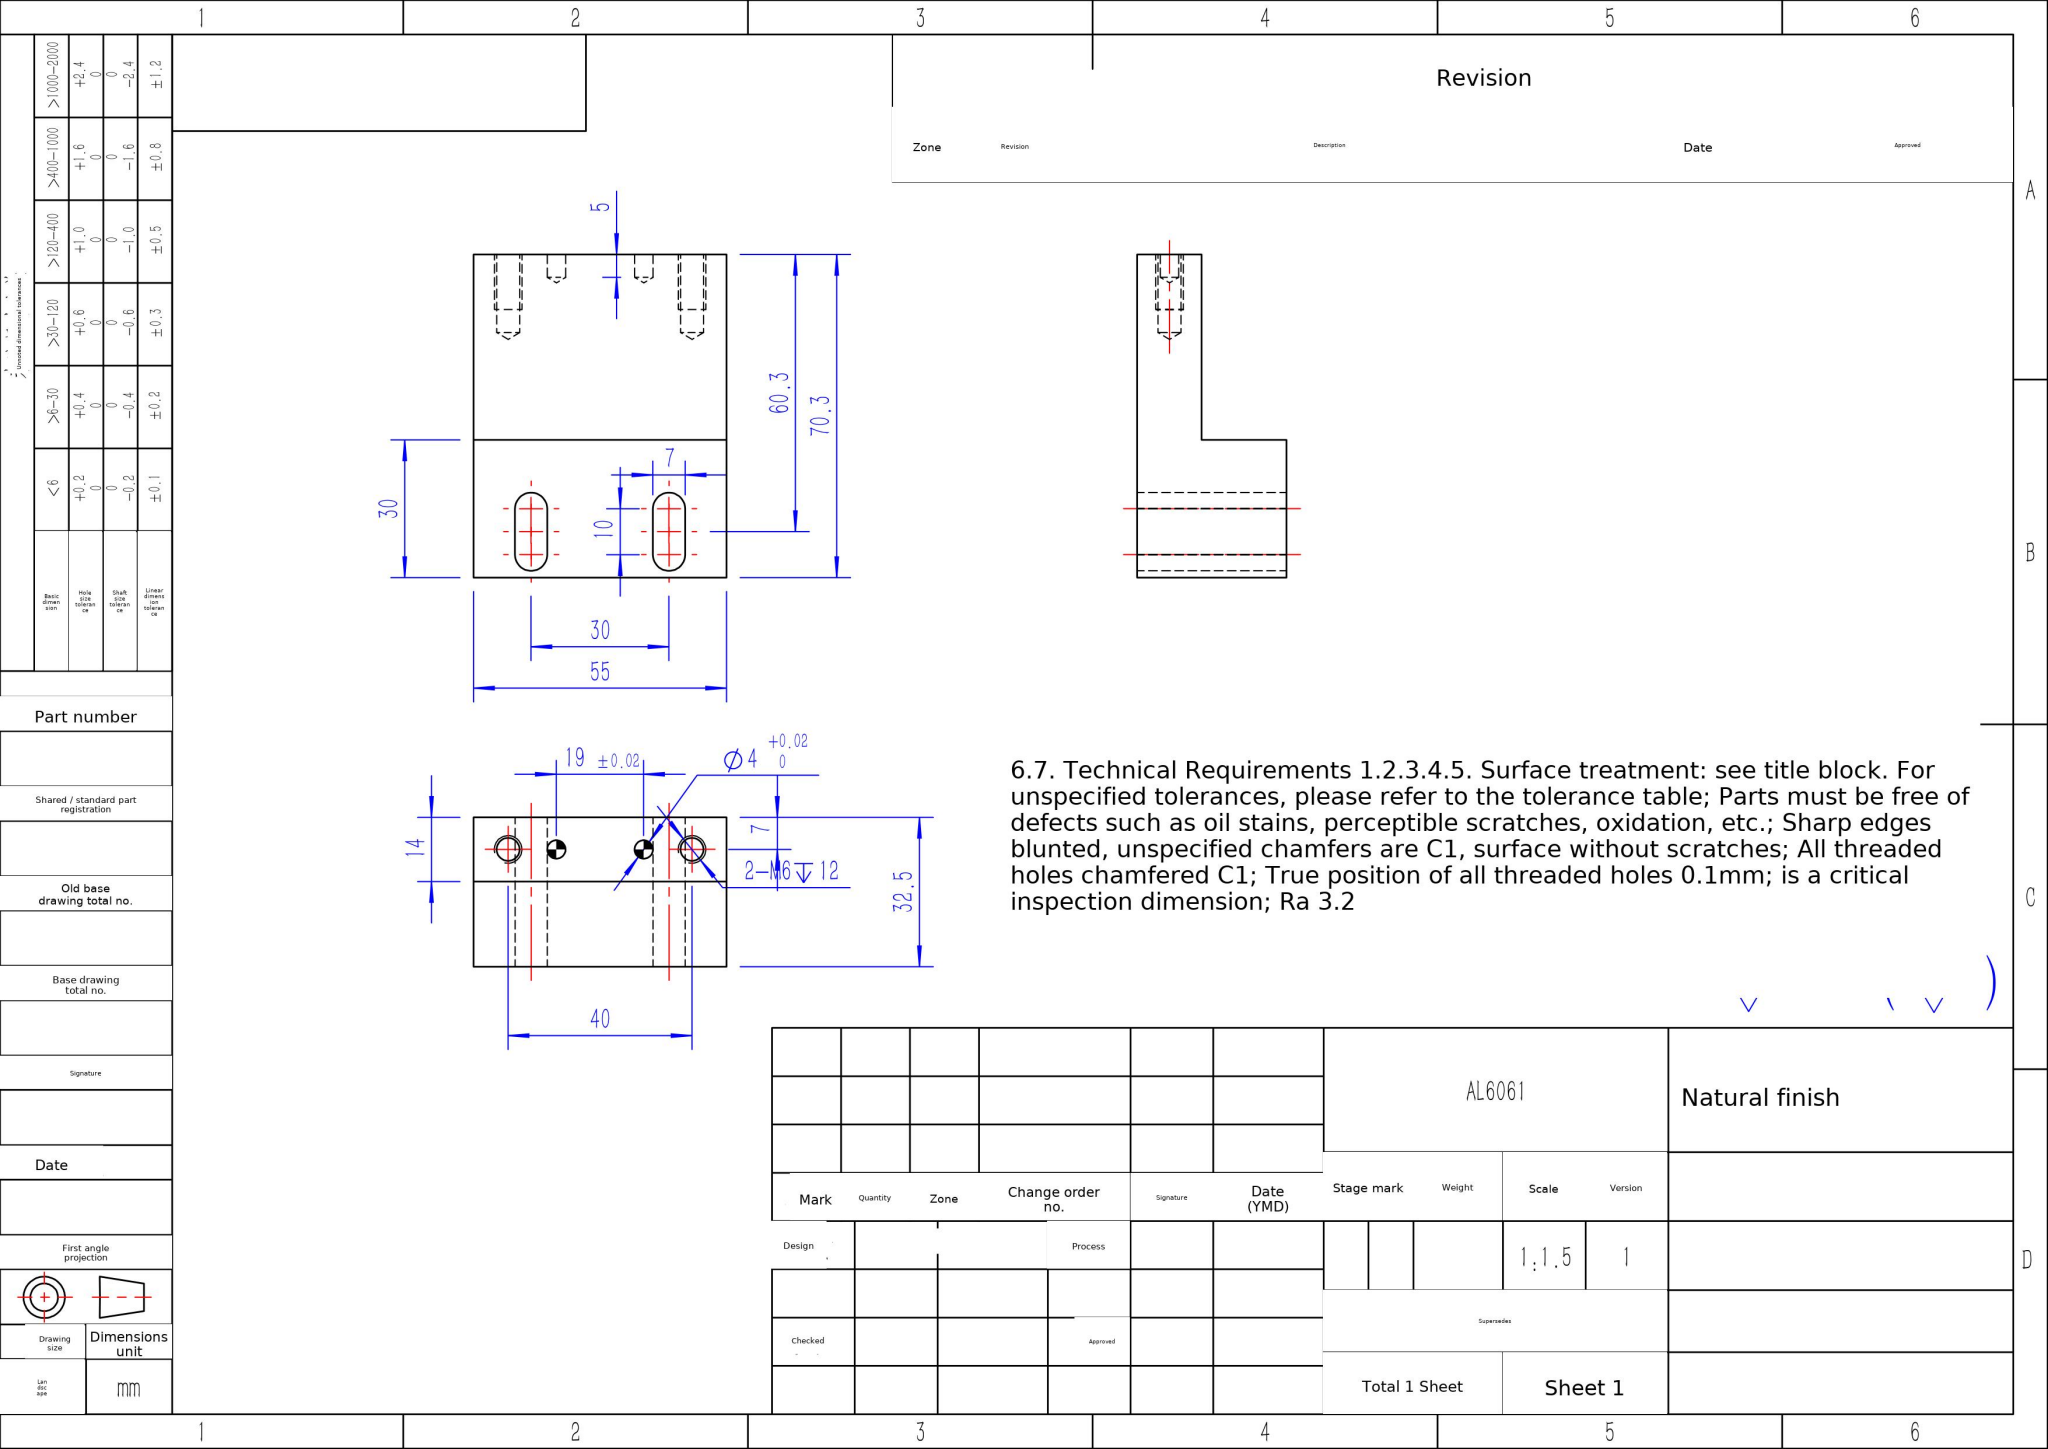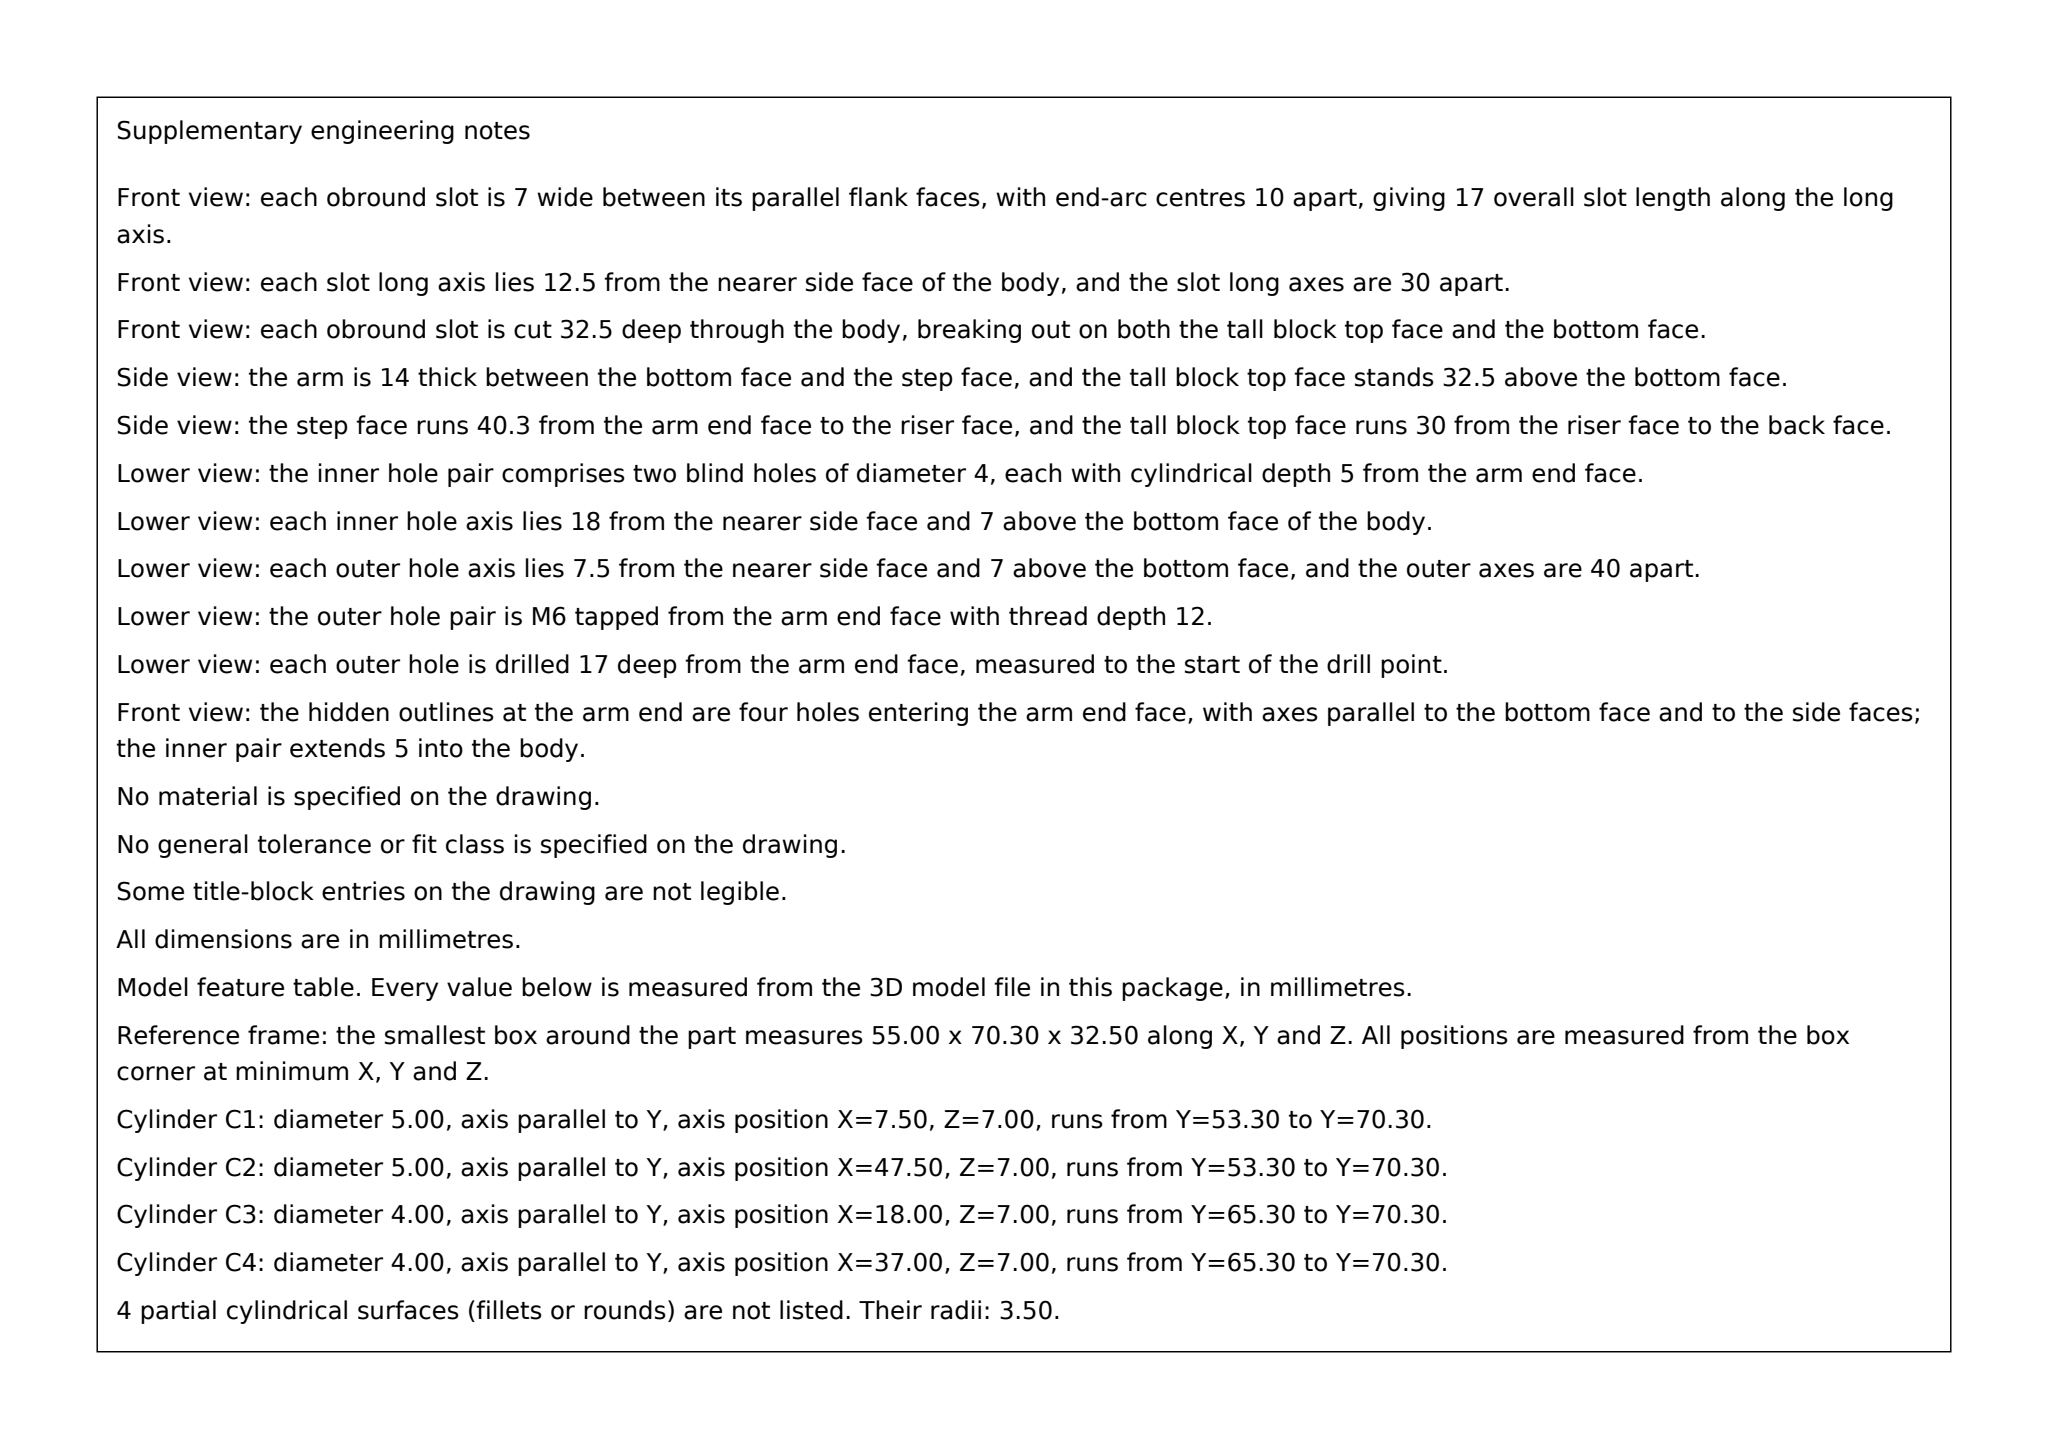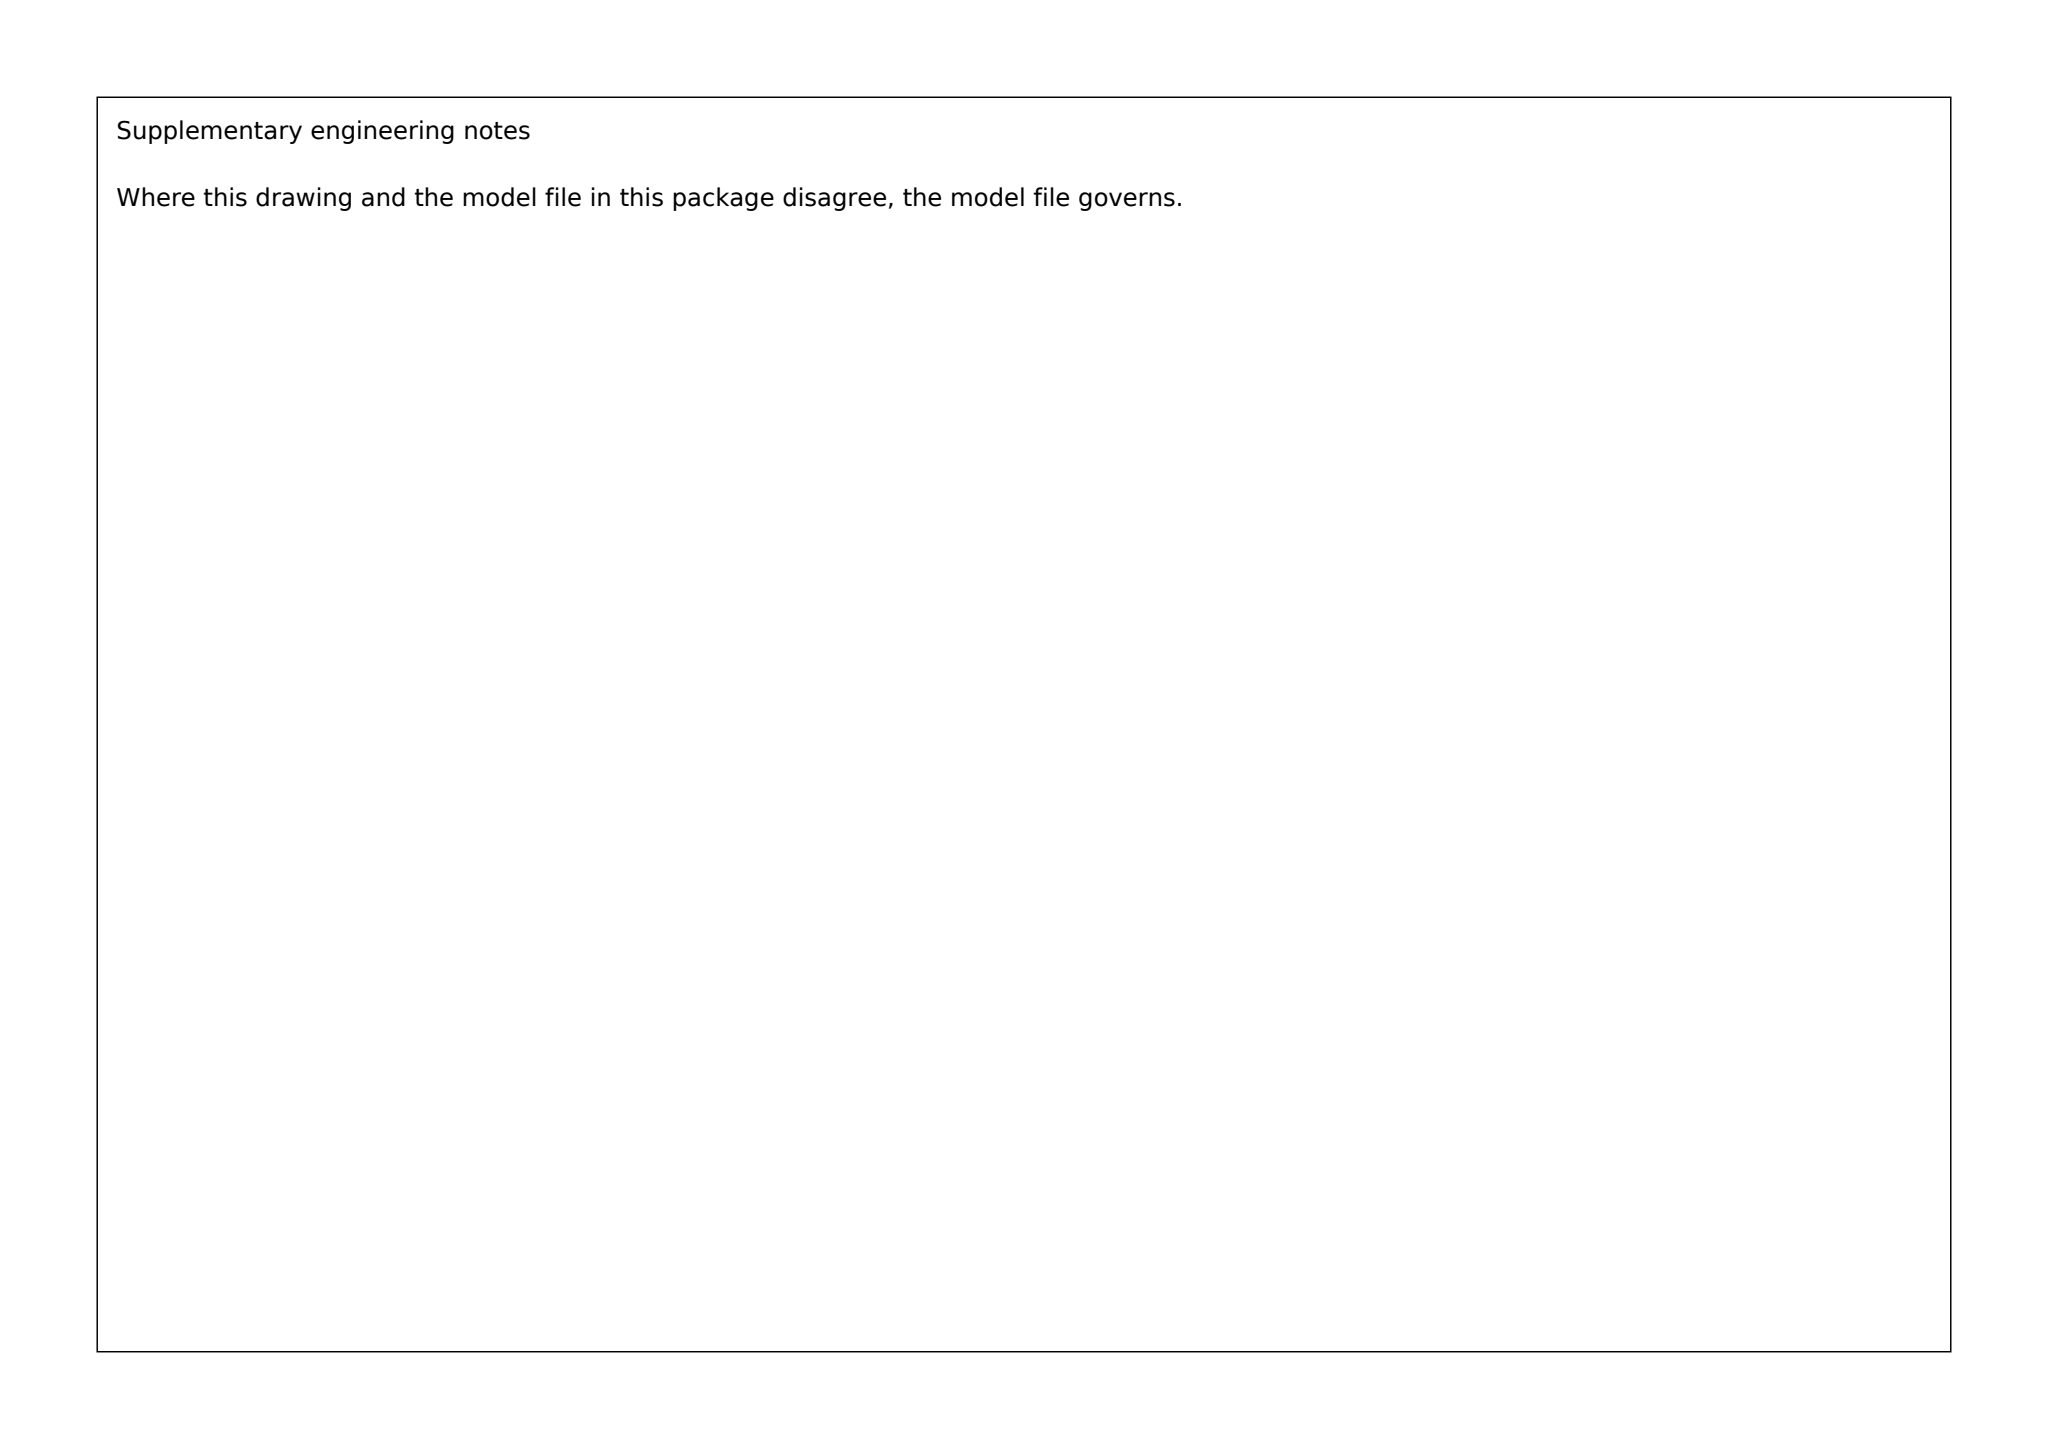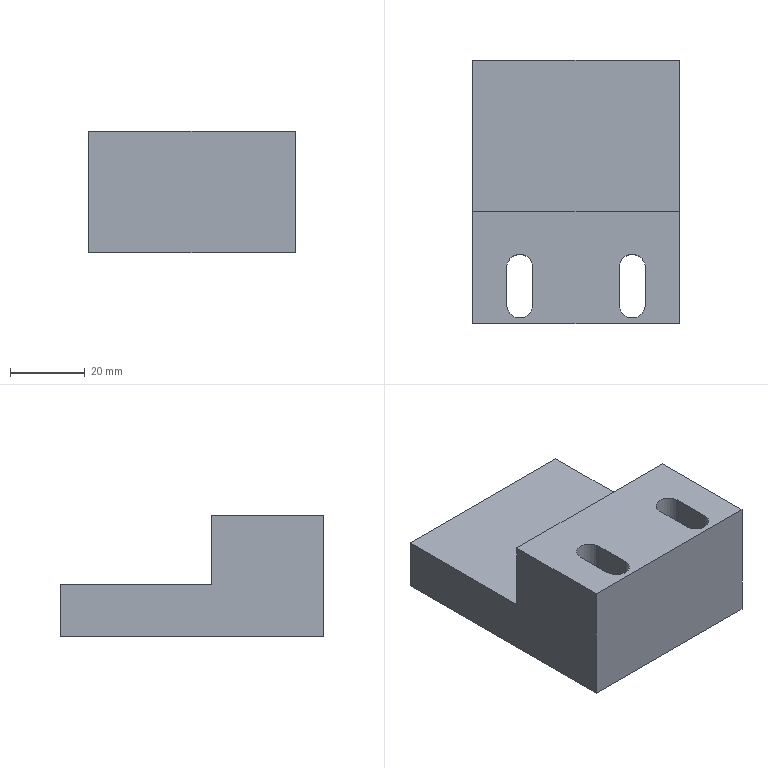Part | SolidWorks | mm | material AL6061 | 1 solid | 32 faces | box 55 x 70.3 x 32.5 mm | volume 76782 mm3 | cylinder 12 | plane 12 | cone 8 | commonest cylinder face diameters 4 x4 5 x4 7 x4
Drawing notes:
2X Ø4 HOLE: 18 FROM LEFT END FACE, SYM ABOUT CL (19 APART) | from the solid: Ø4 cylinders at x=18.0 and x=37.0; bbox x=55.0, so CL=27.5, each 9.5 off CL